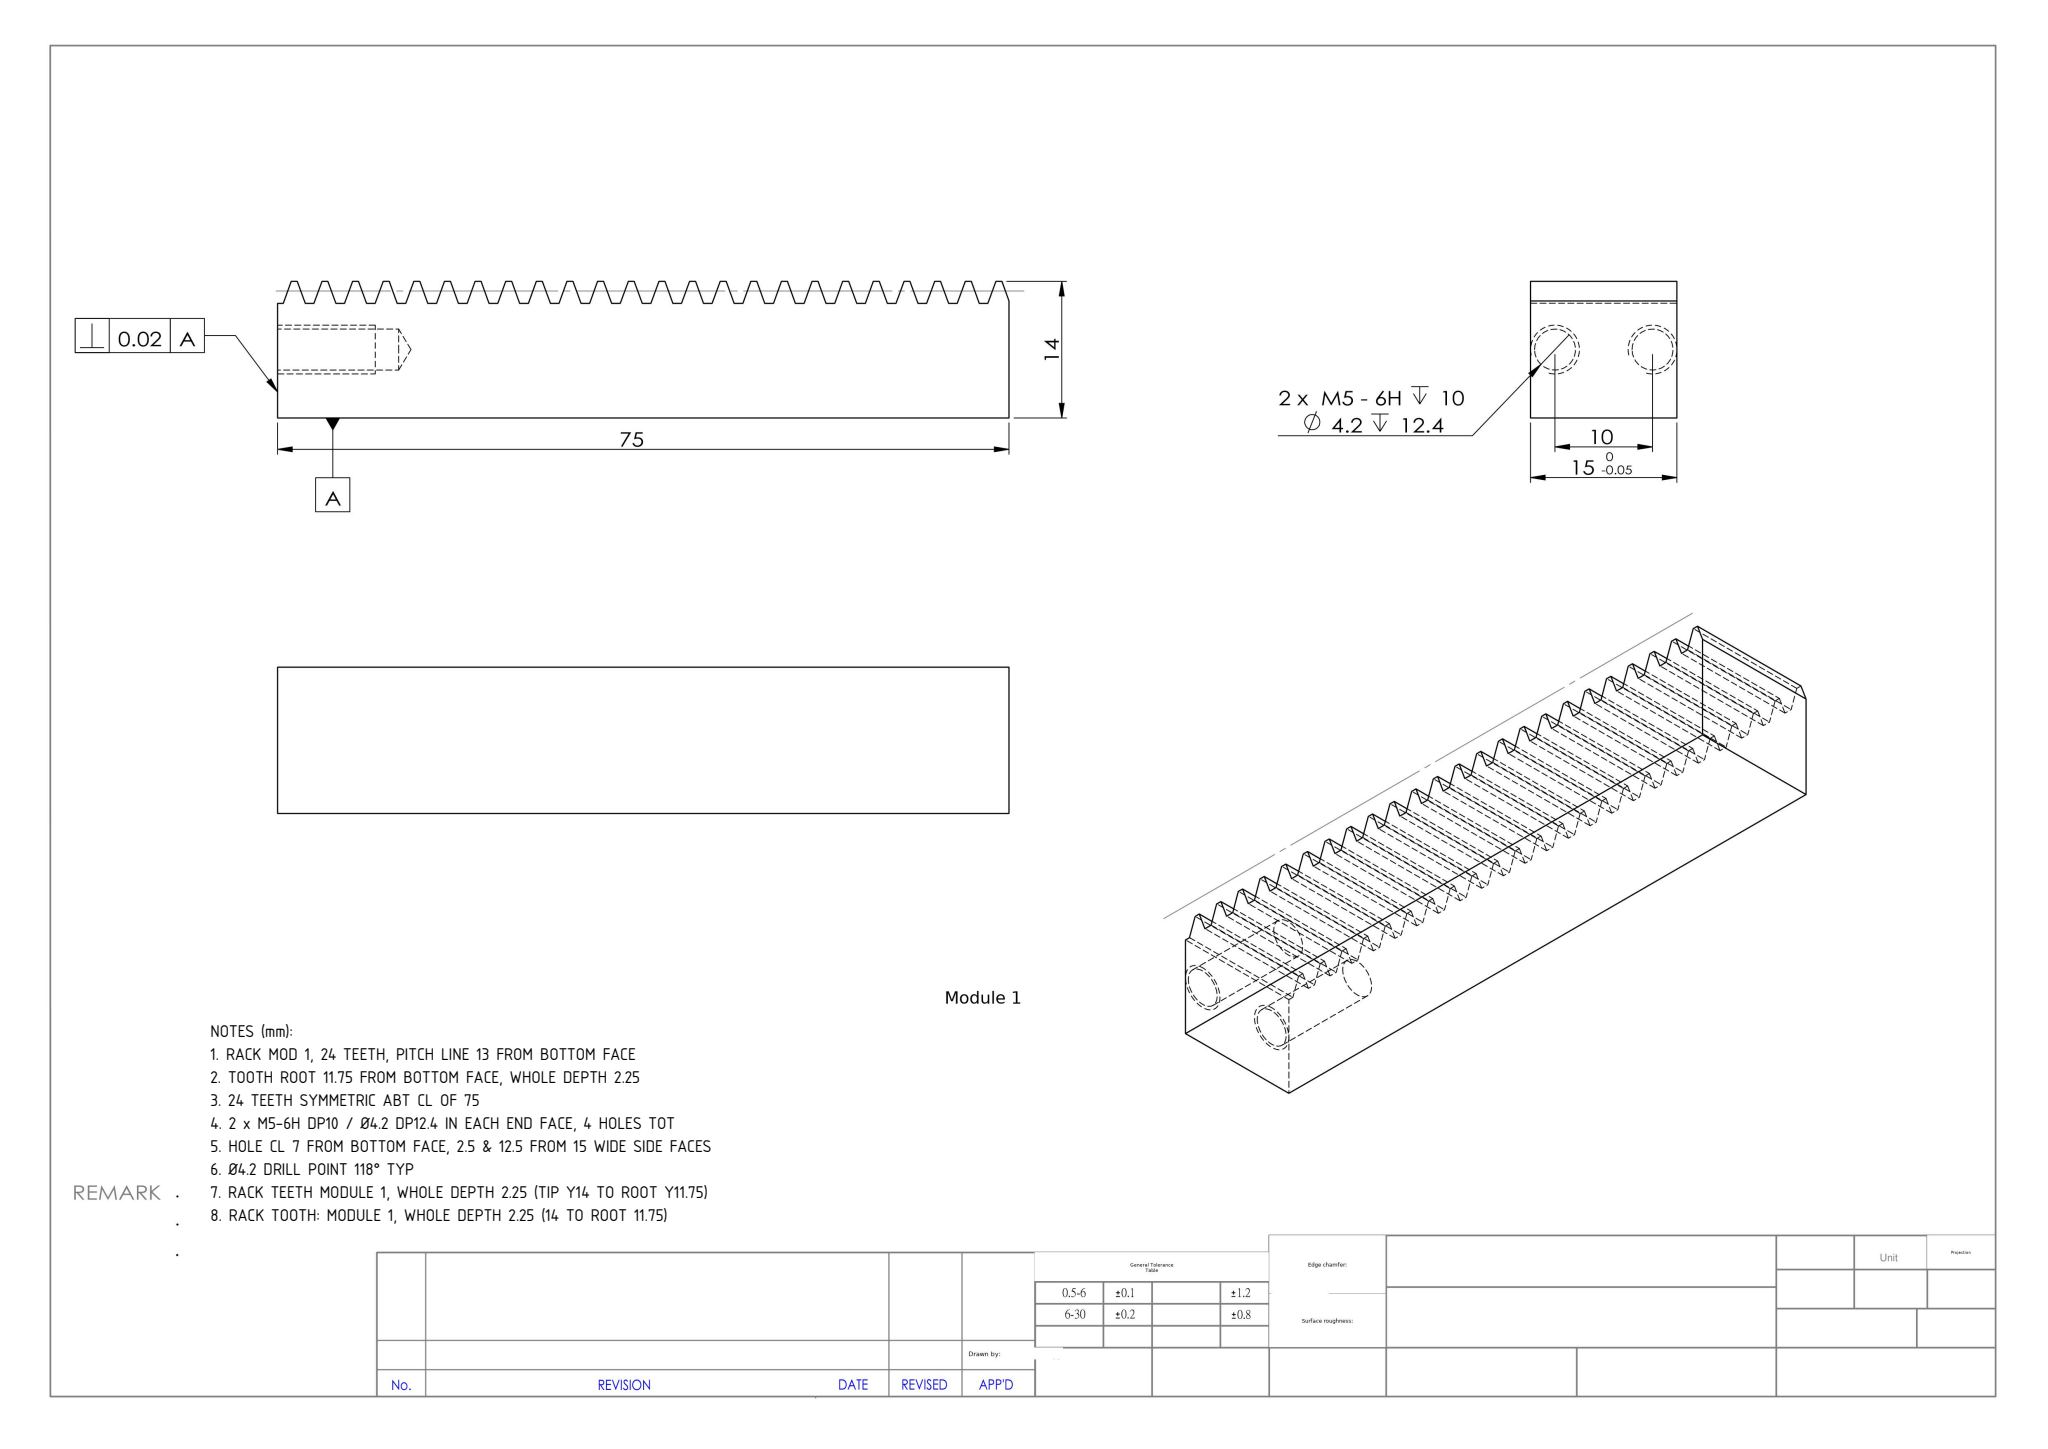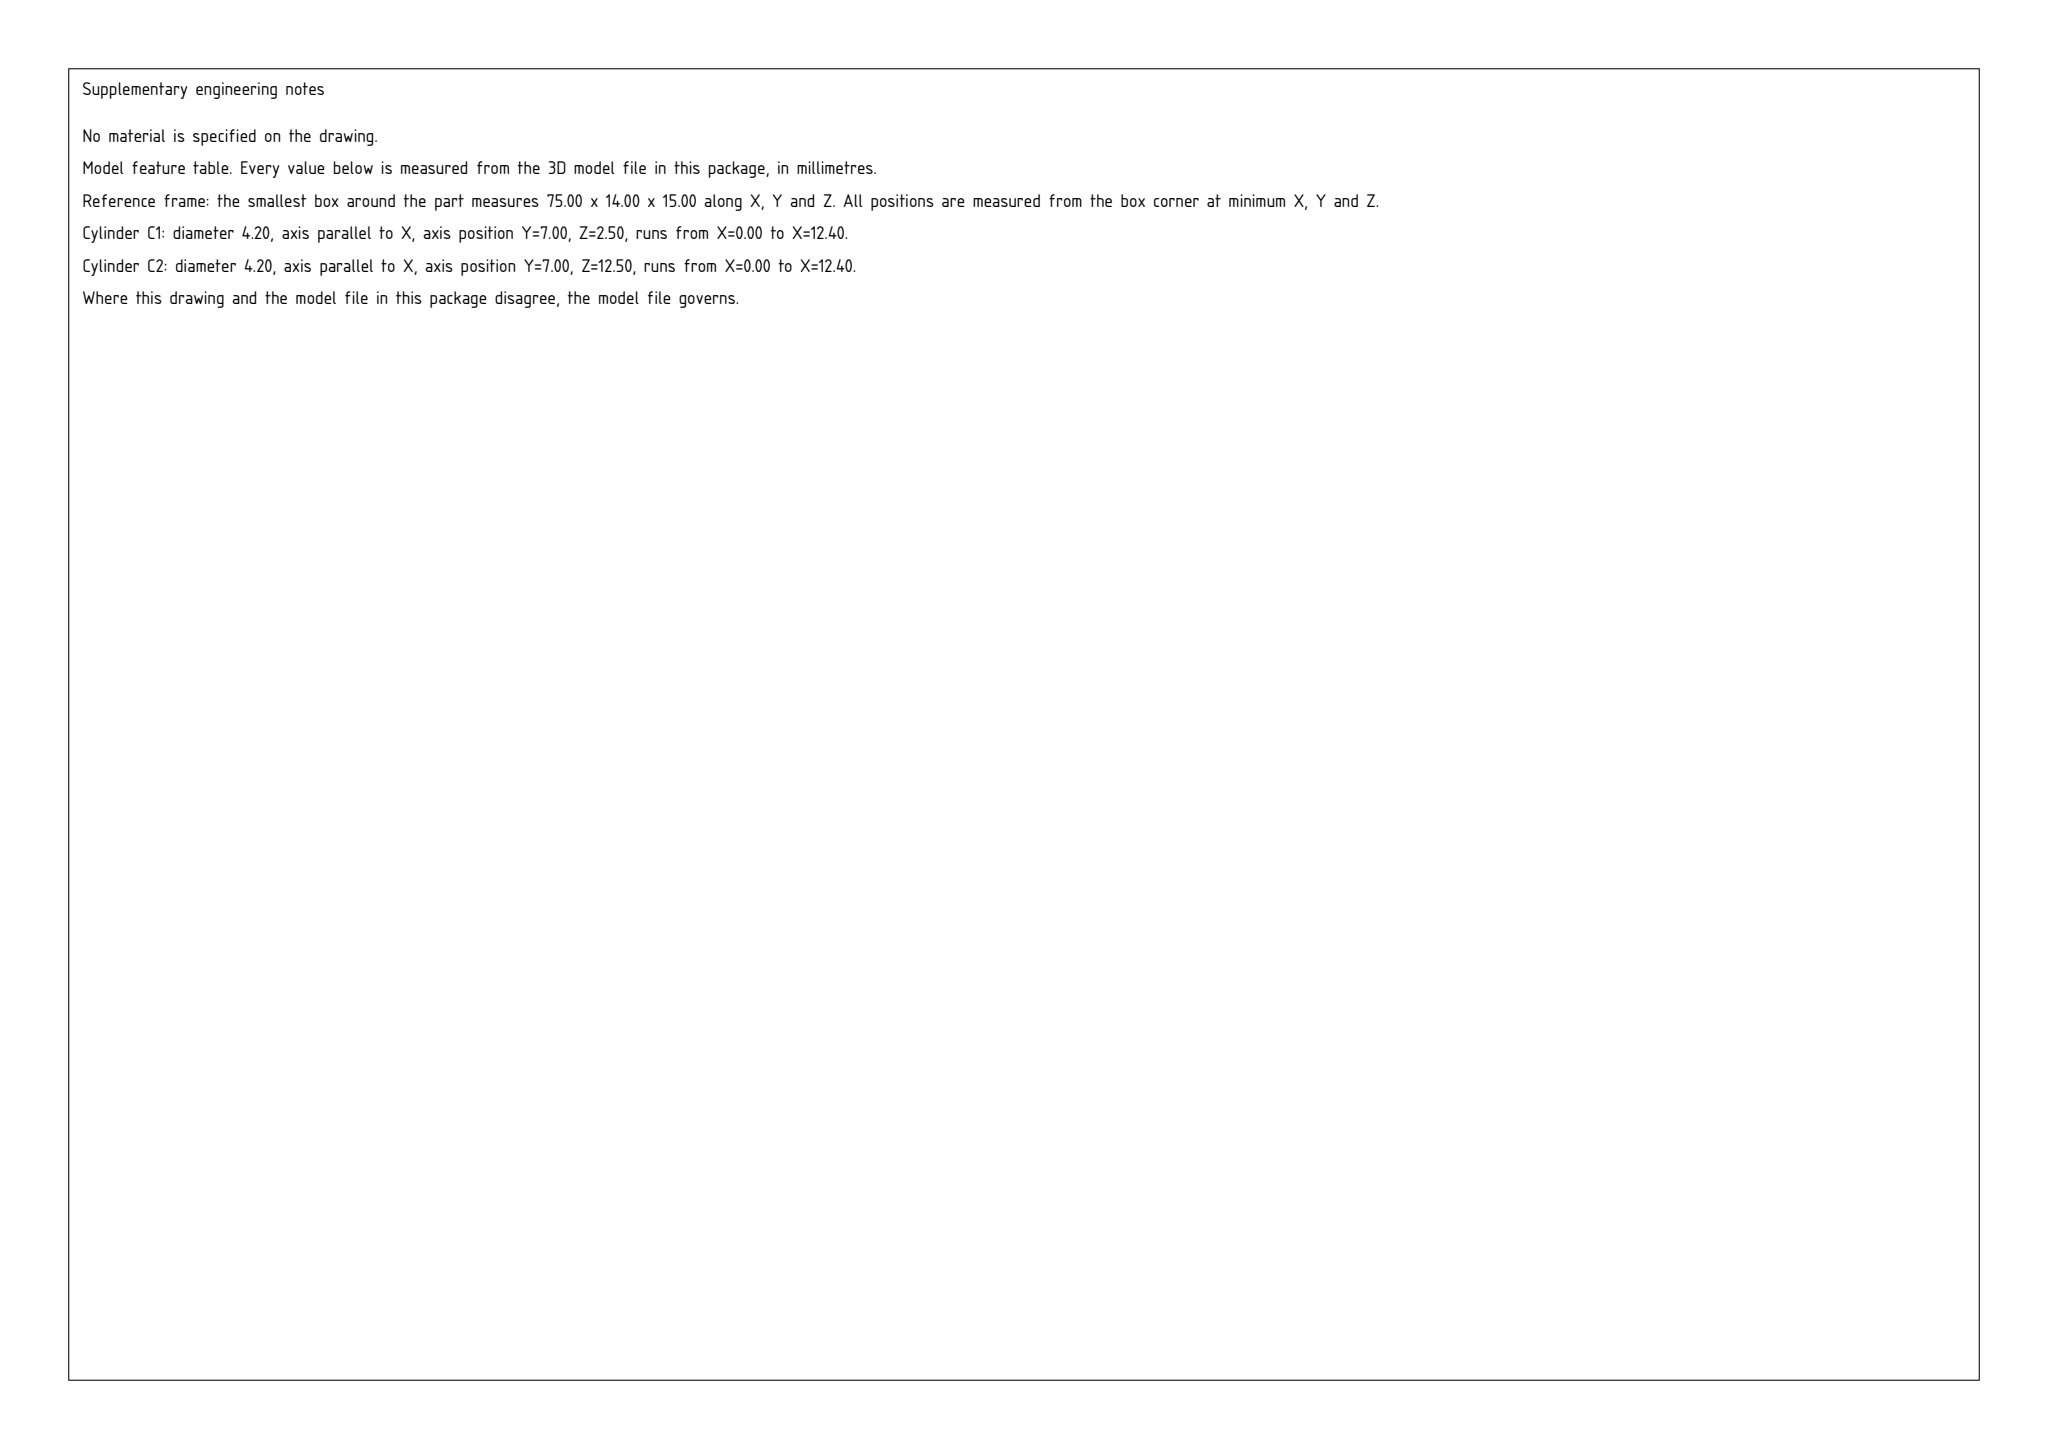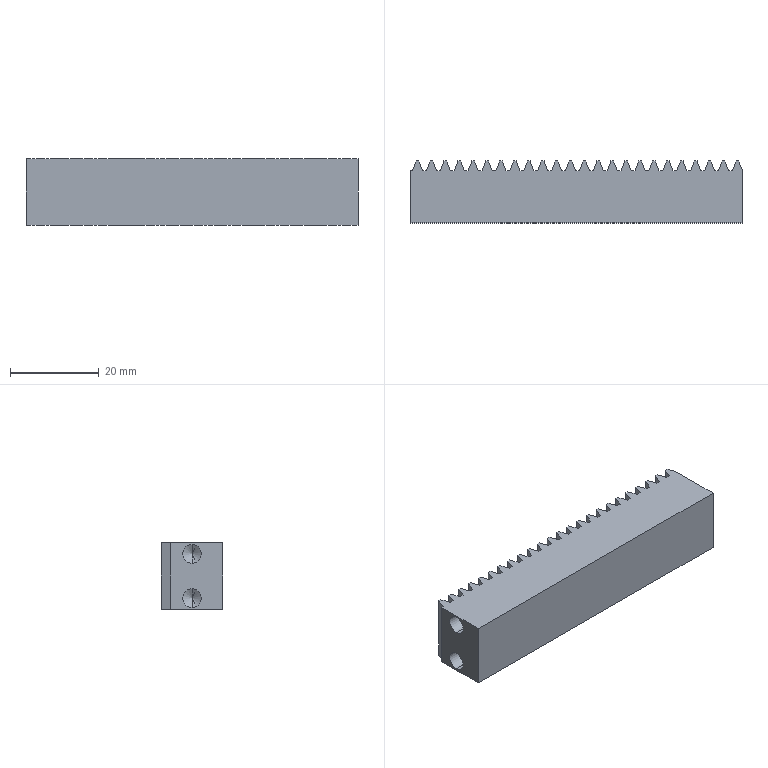Part | SolidWorks | mm | 1 solid | 109 faces | box 75 x 14 x 15 mm | volume 14025 mm3 | plane 101 | cylinder 4 | cone 4 | commonest cylinder face diameters 4.2 x4
Drawing notes:
RACK MOD 1, 24 TEETH, PITCH LINE 13 FROM BOTTOM FACE | from the solid: 24 tip planes y=14.0, 24 root planes y=11.75; tip to pitch 1 (mod 1)
TOOTH ROOT 11.75 FROM BOTTOM FACE, WHOLE DEPTH 2.25 | from the solid: axis_planes y=11.75 (24) and y=14.0 (24)
24 TEETH SYMMETRIC ABT CL OF 75 | from the solid: 24 root/tip planes distributed within bbox x=0..75
2 x M5-6H DP10 / Ø4.2 DP12.4 IN EACH END FACE, 4 HOLES TOT | from the solid: 4.2 dia x-axis cyls, count 2 at z=2.5 and 2 at z=12.5, L=12.4, ends x=0 and x=75
HOLE CL 7 FROM BOTTOM FACE, 2.5 & 12.5 FROM 15 WIDE SIDE FACES | from the solid: cylinders dia 4.2 at y=7.0, z=2.5 and z=12.5; bbox 14 high, 15 wide
Ø4.2 DRILL POINT 118° TYP | from the solid: cones included angle 118.0, ref dia 4.2, qty 4
RACK TEETH MODULE 1, WHOLE DEPTH 2.25 (TIP Y14 TO ROOT Y11.75) | from the solid: axis_planes y=14.0 (24 tip lands) and y=11.75 (24 root lands); 14.0-11.75=2.25 with Module 1 note
RACK TOOTH: MODULE 1, WHOLE DEPTH 2.25 (14 TO ROOT 11.75) | from the solid: y-planes at 11.75 (24 root flats) and 14.0 (24 tip flats) -> 2.25 depth, module 1